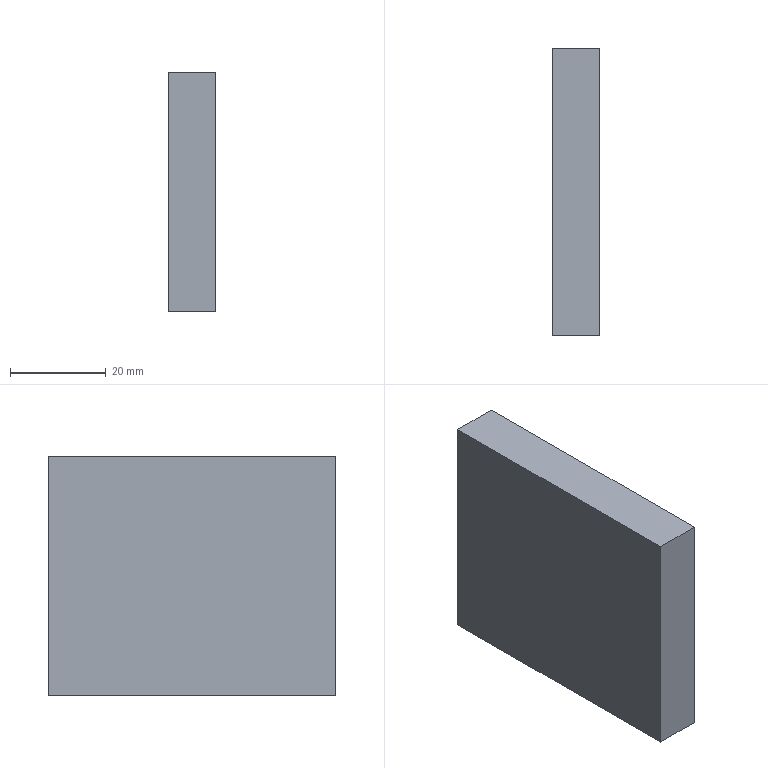Component | SolidWorks | Part4-1 | 1 solid | 6 faces | box 10 x 60 x 50 mm | volume 30000 mm3 | plane 6
build123d program:
from build123d import *

# Parameters (mm, degrees)
SKETCH1_W           = 50
SKETCH1_H           = 60
BOSS_EXTRUDE1_DEPTH = 10


with BuildPart() as part:
    # Sketch1 → Boss-Extrude1 (new body)
    with BuildSketch(Plane(origin=(0, 0, 0), x_dir=(0, 0, -1), z_dir=(1, 0, 0))):
        Rectangle(SKETCH1_W, SKETCH1_H)
    extrude(amount=BOSS_EXTRUDE1_DEPTH)


solid = part.part

# Placed as in the assembly
solid = solid.moved(Location((90.993, 209, -385), (0, 0, 0)))
STEP:
#1=COLOUR_RGB('',0.7922,0.8196,0.9333);
#2=FILL_AREA_STYLE_COLOUR('',#1);
#3=FILL_AREA_STYLE('',(#2));
#4=SURFACE_STYLE_FILL_AREA(#3);
#5=SURFACE_SIDE_STYLE('',(#4));
#6=SURFACE_STYLE_USAGE(.BOTH.,#5);
#7=PRESENTATION_STYLE_ASSIGNMENT((#6));
#8=CARTESIAN_POINT('',(3.582,7.047,-16.142));
#9=VERTEX_POINT('',#8);
#10=CARTESIAN_POINT('',(3.582,9.409,-16.142));
#11=VERTEX_POINT('',#10);
#12=CARTESIAN_POINT('',(3.582,7.047,-16.142));
#13=DIRECTION('',(0.,1.,0.));
#14=VECTOR('',#13,39.37);
#15=LINE('',#12,#14);
#16=EDGE_CURVE('',#9,#11,#15,.T.);
#17=ORIENTED_EDGE('',*,*,#16,.T.);
#18=CARTESIAN_POINT('',(3.976,9.409,-16.142));
#19=VERTEX_POINT('',#18);
#20=CARTESIAN_POINT('',(3.976,9.409,-16.142));
#21=DIRECTION('',(-1.,0.,0.));
#22=VECTOR('',#21,39.37);
#23=LINE('',#20,#22);
#24=EDGE_CURVE('',#19,#11,#23,.T.);
#25=ORIENTED_EDGE('',*,*,#24,.F.);
#26=CARTESIAN_POINT('',(3.976,7.047,-16.142));
#27=VERTEX_POINT('',#26);
#28=CARTESIAN_POINT('',(3.976,7.047,-16.142));
#29=DIRECTION('',(0.,1.,0.));
#30=VECTOR('',#29,39.37);
#31=LINE('',#28,#30);
#32=EDGE_CURVE('',#27,#19,#31,.T.);
#33=ORIENTED_EDGE('',*,*,#32,.F.);
#34=CARTESIAN_POINT('',(3.976,7.047,-16.142));
#35=DIRECTION('',(-1.,0.,0.));
#36=VECTOR('',#35,39.37);
#37=LINE('',#34,#36);
#38=EDGE_CURVE('',#27,#9,#37,.T.);
#39=ORIENTED_EDGE('',*,*,#38,.T.);
#40=EDGE_LOOP('',(#17,#25,#33,#39));
#41=FACE_OUTER_BOUND('',#40,.T.);
#42=CARTESIAN_POINT('',(3.976,7.047,-16.142));
#43=DIRECTION('',(0.,0.,1.));
#44=DIRECTION('',(1.,0.,0.));
#45=AXIS2_PLACEMENT_3D('',#42,#43,#44);
#46=PLANE('',#45);
#47=ADVANCED_FACE('',(#41),#46,.F.);
#48=CARTESIAN_POINT('',(3.582,9.409,-14.173));
#49=VERTEX_POINT('',#48);
#50=CARTESIAN_POINT('',(3.582,9.409,-14.173));
#51=DIRECTION('',(0.,0.,1.));
#52=VECTOR('',#51,39.37);
#53=LINE('',#50,#52);
#54=EDGE_CURVE('',#11,#49,#53,.T.);
#55=ORIENTED_EDGE('',*,*,#54,.T.);
#56=CARTESIAN_POINT('',(3.976,9.409,-14.173));
#57=VERTEX_POINT('',#56);
#58=CARTESIAN_POINT('',(3.976,9.409,-14.173));
#59=DIRECTION('',(-1.,0.,0.));
#60=VECTOR('',#59,39.37);
#61=LINE('',#58,#60);
#62=EDGE_CURVE('',#57,#49,#61,.T.);
#63=ORIENTED_EDGE('',*,*,#62,.F.);
#64=CARTESIAN_POINT('',(3.976,9.409,-14.173));
#65=DIRECTION('',(0.,0.,1.));
#66=VECTOR('',#65,39.37);
#67=LINE('',#64,#66);
#68=EDGE_CURVE('',#19,#57,#67,.T.);
#69=ORIENTED_EDGE('',*,*,#68,.F.);
#70=ORIENTED_EDGE('',*,*,#24,.T.);
#71=EDGE_LOOP('',(#55,#63,#69,#70));
#72=FACE_OUTER_BOUND('',#71,.T.);
#73=CARTESIAN_POINT('',(3.976,9.409,-14.173));
#74=DIRECTION('',(0.,-1.,0.));
#75=DIRECTION('',(0.,0.,-1.));
#76=AXIS2_PLACEMENT_3D('',#73,#74,#75);
#77=PLANE('',#76);
#78=ADVANCED_FACE('',(#72),#77,.F.);
#79=CARTESIAN_POINT('',(3.582,7.047,-14.173));
#80=VERTEX_POINT('',#79);
#81=CARTESIAN_POINT('',(3.582,7.047,-14.173));
#82=DIRECTION('',(0.,-1.,0.));
#83=VECTOR('',#82,39.37);
#84=LINE('',#81,#83);
#85=EDGE_CURVE('',#49,#80,#84,.T.);
#86=ORIENTED_EDGE('',*,*,#85,.T.);
#87=CARTESIAN_POINT('',(3.976,7.047,-14.173));
#88=VERTEX_POINT('',#87);
#89=CARTESIAN_POINT('',(3.976,7.047,-14.173));
#90=DIRECTION('',(-1.,0.,0.));
#91=VECTOR('',#90,39.37);
#92=LINE('',#89,#91);
#93=EDGE_CURVE('',#88,#80,#92,.T.);
#94=ORIENTED_EDGE('',*,*,#93,.F.);
#95=CARTESIAN_POINT('',(3.976,7.047,-14.173));
#96=DIRECTION('',(0.,-1.,0.));
#97=VECTOR('',#96,39.37);
#98=LINE('',#95,#97);
#99=EDGE_CURVE('',#57,#88,#98,.T.);
#100=ORIENTED_EDGE('',*,*,#99,.F.);
#101=ORIENTED_EDGE('',*,*,#62,.T.);
#102=EDGE_LOOP('',(#86,#94,#100,#101));
#103=FACE_OUTER_BOUND('',#102,.T.);
#104=CARTESIAN_POINT('',(3.976,7.047,-14.173));
#105=DIRECTION('',(0.,0.,-1.));
#106=DIRECTION('',(-1.,0.,0.));
#107=AXIS2_PLACEMENT_3D('',#104,#105,#106);
#108=PLANE('',#107);
#109=ADVANCED_FACE('',(#103),#108,.F.);
#110=CARTESIAN_POINT('',(3.582,7.047,-14.173));
#111=DIRECTION('',(0.,0.,-1.));
#112=VECTOR('',#111,39.37);
#113=LINE('',#110,#112);
#114=EDGE_CURVE('',#80,#9,#113,.T.);
#115=ORIENTED_EDGE('',*,*,#114,.T.);
#116=ORIENTED_EDGE('',*,*,#38,.F.);
#117=CARTESIAN_POINT('',(3.976,7.047,-14.173));
#118=DIRECTION('',(0.,0.,-1.));
#119=VECTOR('',#118,39.37);
#120=LINE('',#117,#119);
#121=EDGE_CURVE('',#88,#27,#120,.T.);
#122=ORIENTED_EDGE('',*,*,#121,.F.);
#123=ORIENTED_EDGE('',*,*,#93,.T.);
#124=EDGE_LOOP('',(#115,#116,#122,#123));
#125=FACE_OUTER_BOUND('',#124,.T.);
#126=CARTESIAN_POINT('',(3.976,7.047,-14.173));
#127=DIRECTION('',(0.,1.,0.));
#128=DIRECTION('',(0.,0.,1.));
#129=AXIS2_PLACEMENT_3D('',#126,#127,#128);
#130=PLANE('',#129);
#131=ADVANCED_FACE('',(#125),#130,.F.);
#132=ORIENTED_EDGE('',*,*,#32,.T.);
#133=ORIENTED_EDGE('',*,*,#68,.T.);
#134=ORIENTED_EDGE('',*,*,#99,.T.);
#135=ORIENTED_EDGE('',*,*,#121,.T.);
#136=EDGE_LOOP('',(#132,#133,#134,#135));
#137=FACE_OUTER_BOUND('',#136,.T.);
#138=CARTESIAN_POINT('',(3.976,8.228,-15.157));
#139=DIRECTION('',(-1.,0.,0.));
#140=DIRECTION('',(0.,0.,1.));
#141=AXIS2_PLACEMENT_3D('',#138,#139,#140);
#142=PLANE('',#141);
#143=ADVANCED_FACE('',(#137),#142,.F.);
#144=ORIENTED_EDGE('',*,*,#16,.F.);
#145=ORIENTED_EDGE('',*,*,#114,.F.);
#146=ORIENTED_EDGE('',*,*,#85,.F.);
#147=ORIENTED_EDGE('',*,*,#54,.F.);
#148=EDGE_LOOP('',(#144,#145,#146,#147));
#149=FACE_OUTER_BOUND('',#148,.T.);
#150=CARTESIAN_POINT('',(3.582,8.228,-15.157));
#151=DIRECTION('',(-1.,0.,0.));
#152=DIRECTION('',(0.,0.,1.));
#153=AXIS2_PLACEMENT_3D('',#150,#151,#152);
#154=PLANE('',#153);
#155=ADVANCED_FACE('',(#149),#154,.T.);
#156=CLOSED_SHELL('',(#47,#78,#109,#131,#143,#155));
#157=MANIFOLD_SOLID_BREP('',#156);
#158=STYLED_ITEM('',(#7),#157);
#159=(LENGTH_UNIT()NAMED_UNIT(*)SI_UNIT($,.METRE.));
#160=LENGTH_MEASURE_WITH_UNIT(LENGTH_MEASURE(0.0254),#159);
#161=DIMENSIONAL_EXPONENTS(1.,0.,0.,0.,0.,0.,0.);
#162=(CONVERSION_BASED_UNIT('',#160)LENGTH_UNIT()NAMED_UNIT(#161));
#163=UNCERTAINTY_MEASURE_WITH_UNIT(LENGTH_MEASURE(0.00001),#162,'','');
#164=(NAMED_UNIT(*)PLANE_ANGLE_UNIT()SI_UNIT($,.RADIAN.));
#165=(NAMED_UNIT(*)SI_UNIT($,.STERADIAN.)SOLID_ANGLE_UNIT());
#166=(GEOMETRIC_REPRESENTATION_CONTEXT(3)GLOBAL_UNCERTAINTY_ASSIGNED_CONTEXT((#163))GLOBAL_UNIT_ASSIGNED_CONTEXT((#162,#164,#165))REPRESENTATION_CONTEXT('',''));
#167=MECHANICAL_DESIGN_GEOMETRIC_PRESENTATION_REPRESENTATION('',(#158),#166);
#168=PRESENTATION_LAYER_ASSIGNMENT('','',(#158));
#169=CARTESIAN_POINT('',(0.,0.,0.));
#170=DIRECTION('',(0.,0.,1.));
#171=DIRECTION('',(1.,0.,0.));
#172=AXIS2_PLACEMENT_3D('',#169,#170,#171);
#173=(LENGTH_UNIT()NAMED_UNIT(*)SI_UNIT($,.METRE.));
#174=LENGTH_MEASURE_WITH_UNIT(LENGTH_MEASURE(0.0254),#173);
#175=DIMENSIONAL_EXPONENTS(1.,0.,0.,0.,0.,0.,0.);
#176=(CONVERSION_BASED_UNIT('',#174)LENGTH_UNIT()NAMED_UNIT(#175));
#177=UNCERTAINTY_MEASURE_WITH_UNIT(LENGTH_MEASURE(0.00001),#176,'','');
#178=(NAMED_UNIT(*)PLANE_ANGLE_UNIT()SI_UNIT($,.RADIAN.));
#179=(NAMED_UNIT(*)SI_UNIT($,.STERADIAN.)SOLID_ANGLE_UNIT());
#180=(GEOMETRIC_REPRESENTATION_CONTEXT(3)GLOBAL_UNCERTAINTY_ASSIGNED_CONTEXT((#177))GLOBAL_UNIT_ASSIGNED_CONTEXT((#176,#178,#179))REPRESENTATION_CONTEXT('',''));
#181=ADVANCED_BREP_SHAPE_REPRESENTATION('',(#157,#172),#180);